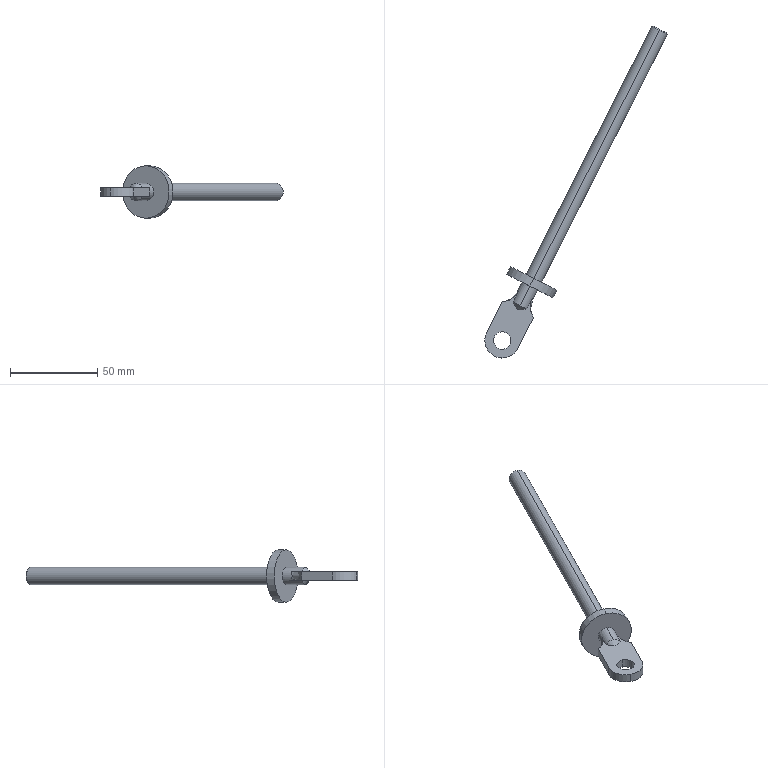Component | SolidWorks | FilmPressingSoilCoveringMechanism2Reverse-2_TieRod2-1 | 1 solid | 24 faces | box 104.65 x 190.43 x 30 mm | volume 19756 mm3 | cylinder 10 | plane 7 | cone 5 | spline 2 | commonest cylinder face diameters 10 x6 30 x2 20 x2
STEP:
#1=COLOUR_RGB('',0.7922,0.8196,0.9333);
#2=FILL_AREA_STYLE_COLOUR('',#1);
#3=FILL_AREA_STYLE('',(#2));
#4=SURFACE_STYLE_FILL_AREA(#3);
#5=SURFACE_SIDE_STYLE('',(#4));
#6=SURFACE_STYLE_USAGE(.BOTH.,#5);
#7=PRESENTATION_STYLE_ASSIGNMENT((#6));
#8=CARTESIAN_POINT('',(-66.242,-3.201,100.924));
#9=VERTEX_POINT('',#8);
#10=CARTESIAN_POINT('',(-66.242,-3.201,101.278));
#11=VERTEX_POINT('',#10);
#12=CARTESIAN_POINT('',(-66.242,-3.201,101.101));
#13=DIRECTION('',(0.4521,0.892,0.));
#14=DIRECTION('',(0.,0.,-1.));
#15=AXIS2_PLACEMENT_3D('',#12,#13,#14);
#16=CIRCLE('',#15,0.1772);
#17=EDGE_CURVE('',#9,#11,#16,.T.);
#18=ORIENTED_EDGE('',*,*,#17,.F.);
#19=CARTESIAN_POINT('',(-66.251,-3.218,100.904));
#20=VERTEX_POINT('',#19);
#21=CARTESIAN_POINT('',(-66.242,-3.201,100.924));
#22=DIRECTION('',(-0.3197,-0.6307,-0.7071));
#23=VECTOR('',#22,39.37);
#24=LINE('',#21,#23);
#25=EDGE_CURVE('',#9,#20,#24,.T.);
#26=ORIENTED_EDGE('',*,*,#25,.T.);
#27=CARTESIAN_POINT('',(-66.251,-3.218,101.298));
#28=VERTEX_POINT('',#27);
#29=CARTESIAN_POINT('',(-66.251,-3.218,101.101));
#30=DIRECTION('',(-0.4521,-0.892,-0.));
#31=DIRECTION('',(0.,0.,-1.));
#32=AXIS2_PLACEMENT_3D('',#29,#30,#31);
#33=CIRCLE('',#32,0.1969);
#34=EDGE_CURVE('',#28,#20,#33,.T.);
#35=ORIENTED_EDGE('',*,*,#34,.F.);
#36=CARTESIAN_POINT('',(-66.242,-3.201,101.278));
#37=DIRECTION('',(-0.3197,-0.6307,0.7071));
#38=VECTOR('',#37,39.37);
#39=LINE('',#36,#38);
#40=EDGE_CURVE('',#11,#28,#39,.T.);
#41=ORIENTED_EDGE('',*,*,#40,.F.);
#42=EDGE_LOOP('',(#18,#26,#35,#41));
#43=FACE_OUTER_BOUND('',#42,.T.);
#44=CARTESIAN_POINT('',(-66.242,-3.201,101.101));
#45=DIRECTION('',(-0.4521,-0.892,-0.));
#46=DIRECTION('',(-0.,-0.,1.));
#47=AXIS2_PLACEMENT_3D('',#44,#45,#46);
#48=CONICAL_SURFACE('',#47,0.1772,0.7854);
#49=ADVANCED_FACE('',(#43),#48,.T.);
#50=CARTESIAN_POINT('',(-69.446,-9.522,101.003));
#51=VERTEX_POINT('',#50);
#52=CARTESIAN_POINT('',(-69.25,-9.511,101.003));
#53=VERTEX_POINT('',#52);
#54=CARTESIAN_POINT('',(-69.446,-9.522,101.003));
#55=CARTESIAN_POINT('',(-69.439,-9.526,101.003));
#56=CARTESIAN_POINT('',(-69.431,-9.528,101.003));
#57=CARTESIAN_POINT('',(-69.415,-9.532,101.003));
#58=CARTESIAN_POINT('',(-69.406,-9.533,101.003));
#59=CARTESIAN_POINT('',(-69.381,-9.534,101.003));
#60=CARTESIAN_POINT('',(-69.364,-9.533,101.003));
#61=CARTESIAN_POINT('',(-69.331,-9.529,101.003));
#62=CARTESIAN_POINT('',(-69.315,-9.526,101.003));
#63=CARTESIAN_POINT('',(-69.282,-9.519,101.003));
#64=CARTESIAN_POINT('',(-69.266,-9.515,101.003));
#65=CARTESIAN_POINT('',(-69.25,-9.511,101.003));
#66=B_SPLINE_CURVE_WITH_KNOTS('',3,(#54,#55,#56,#57,#58,#59,#60,#61,#62,#63,#64,#65),.UNSPECIFIED.,.F.,.F.,(4,2,2,2,2,4),(0.005096,0.005734,0.006372,0.007648,0.008924,0.0102),.UNSPECIFIED.);
#67=EDGE_CURVE('',#51,#53,#66,.T.);
#68=ORIENTED_EDGE('',*,*,#67,.F.);
#69=CARTESIAN_POINT('',(-69.402,-9.434,100.904));
#70=VERTEX_POINT('',#69);
#71=CARTESIAN_POINT('',(-69.402,-9.434,100.904));
#72=DIRECTION('',(0.3197,0.6307,-0.7071));
#73=VECTOR('',#72,39.37);
#74=LINE('',#71,#73);
#75=EDGE_CURVE('',#51,#70,#74,.T.);
#76=ORIENTED_EDGE('',*,*,#75,.T.);
#77=CARTESIAN_POINT('',(-69.402,-9.434,101.101));
#78=DIRECTION('',(0.4521,0.892,0.));
#79=DIRECTION('',(0.,0.,-1.));
#80=AXIS2_PLACEMENT_3D('',#77,#78,#79);
#81=CIRCLE('',#80,0.1969);
#82=EDGE_CURVE('',#53,#70,#81,.T.);
#83=ORIENTED_EDGE('',*,*,#82,.F.);
#84=EDGE_LOOP('',(#68,#76,#83));
#85=FACE_OUTER_BOUND('',#84,.T.);
#86=CARTESIAN_POINT('',(-69.402,-9.434,101.101));
#87=DIRECTION('',(0.4521,0.892,0.));
#88=DIRECTION('',(0.,0.,-1.));
#89=AXIS2_PLACEMENT_3D('',#86,#87,#88);
#90=CONICAL_SURFACE('',#89,0.1969,0.7854);
#91=ADVANCED_FACE('',(#85),#90,.T.);
#92=CARTESIAN_POINT('',(-69.891,-10.4,101.003));
#93=VERTEX_POINT('',#92);
#94=CARTESIAN_POINT('',(-69.713,-10.048,101.003));
#95=VERTEX_POINT('',#94);
#96=CARTESIAN_POINT('',(-69.802,-10.224,101.003));
#97=DIRECTION('',(-0.,-0.,1.));
#98=DIRECTION('',(0.4521,0.892,0.));
#99=AXIS2_PLACEMENT_3D('',#96,#97,#98);
#100=CIRCLE('',#99,0.1969);
#101=EDGE_CURVE('',#93,#95,#100,.T.);
#102=ORIENTED_EDGE('',*,*,#101,.F.);
#103=CARTESIAN_POINT('',(-69.891,-10.4,101.2));
#104=VERTEX_POINT('',#103);
#105=CARTESIAN_POINT('',(-69.891,-10.4,100.019));
#106=DIRECTION('',(-0.,-0.,1.));
#107=VECTOR('',#106,39.37);
#108=LINE('',#105,#107);
#109=EDGE_CURVE('',#93,#104,#108,.T.);
#110=ORIENTED_EDGE('',*,*,#109,.T.);
#111=CARTESIAN_POINT('',(-69.713,-10.048,101.2));
#112=VERTEX_POINT('',#111);
#113=CARTESIAN_POINT('',(-69.802,-10.224,101.2));
#114=DIRECTION('',(-0.,-0.,1.));
#115=DIRECTION('',(0.4521,0.892,0.));
#116=AXIS2_PLACEMENT_3D('',#113,#114,#115);
#117=CIRCLE('',#116,0.1969);
#118=EDGE_CURVE('',#104,#112,#117,.T.);
#119=ORIENTED_EDGE('',*,*,#118,.T.);
#120=CARTESIAN_POINT('',(-69.713,-10.048,100.019));
#121=DIRECTION('',(-0.,-0.,1.));
#122=VECTOR('',#121,39.37);
#123=LINE('',#120,#122);
#124=EDGE_CURVE('',#95,#112,#123,.T.);
#125=ORIENTED_EDGE('',*,*,#124,.F.);
#126=EDGE_LOOP('',(#102,#110,#119,#125));
#127=FACE_OUTER_BOUND('',#126,.T.);
#128=CARTESIAN_POINT('',(-69.802,-10.224,100.019));
#129=DIRECTION('',(-0.,-0.,1.));
#130=DIRECTION('',(0.4521,0.892,0.));
#131=AXIS2_PLACEMENT_3D('',#128,#129,#130);
#132=CYLINDRICAL_SURFACE('',#131,0.1969);
#133=ADVANCED_FACE('',(#127),#132,.F.);
#134=ORIENTED_EDGE('',*,*,#34,.T.);
#135=CARTESIAN_POINT('',(-69.09,-8.819,100.904));
#136=VERTEX_POINT('',#135);
#137=CARTESIAN_POINT('',(-66.242,-3.201,100.904));
#138=DIRECTION('',(-0.4521,-0.892,-0.));
#139=VECTOR('',#138,39.37);
#140=LINE('',#137,#139);
#141=EDGE_CURVE('',#20,#136,#140,.T.);
#142=ORIENTED_EDGE('',*,*,#141,.T.);
#143=CARTESIAN_POINT('',(-69.09,-8.819,101.298));
#144=VERTEX_POINT('',#143);
#145=CARTESIAN_POINT('',(-69.09,-8.819,101.101));
#146=DIRECTION('',(-0.4521,-0.892,-0.));
#147=DIRECTION('',(-0.,-0.,1.));
#148=AXIS2_PLACEMENT_3D('',#145,#146,#147);
#149=CIRCLE('',#148,0.1969);
#150=EDGE_CURVE('',#144,#136,#149,.T.);
#151=ORIENTED_EDGE('',*,*,#150,.F.);
#152=CARTESIAN_POINT('',(-66.242,-3.201,101.298));
#153=DIRECTION('',(-0.4521,-0.892,-0.));
#154=VECTOR('',#153,39.37);
#155=LINE('',#152,#154);
#156=EDGE_CURVE('',#28,#144,#155,.T.);
#157=ORIENTED_EDGE('',*,*,#156,.F.);
#158=EDGE_LOOP('',(#134,#142,#151,#157));
#159=FACE_OUTER_BOUND('',#158,.T.);
#160=CARTESIAN_POINT('',(-66.242,-3.201,101.101));
#161=DIRECTION('',(-0.4521,-0.892,-0.));
#162=DIRECTION('',(-0.,-0.,1.));
#163=AXIS2_PLACEMENT_3D('',#160,#161,#162);
#164=CYLINDRICAL_SURFACE('',#163,0.1969);
#165=ADVANCED_FACE('',(#159),#164,.T.);
#166=CARTESIAN_POINT('',(-69.179,-8.995,101.692));
#167=VERTEX_POINT('',#166);
#168=CARTESIAN_POINT('',(-69.179,-8.995,100.511));
#169=VERTEX_POINT('',#168);
#170=CARTESIAN_POINT('',(-69.179,-8.995,101.101));
#171=DIRECTION('',(-0.4521,-0.892,-0.));
#172=DIRECTION('',(-0.,-0.,1.));
#173=AXIS2_PLACEMENT_3D('',#170,#171,#172);
#174=CIRCLE('',#173,0.5906);
#175=EDGE_CURVE('',#167,#169,#174,.T.);
#176=ORIENTED_EDGE('',*,*,#175,.F.);
#177=CARTESIAN_POINT('',(-69.09,-8.819,101.692));
#178=VERTEX_POINT('',#177);
#179=CARTESIAN_POINT('',(-69.179,-8.995,101.692));
#180=DIRECTION('',(0.4521,0.892,0.));
#181=VECTOR('',#180,39.37);
#182=LINE('',#179,#181);
#183=EDGE_CURVE('',#167,#178,#182,.T.);
#184=ORIENTED_EDGE('',*,*,#183,.T.);
#185=CARTESIAN_POINT('',(-69.09,-8.819,100.511));
#186=VERTEX_POINT('',#185);
#187=CARTESIAN_POINT('',(-69.09,-8.819,101.101));
#188=DIRECTION('',(-0.4521,-0.892,-0.));
#189=DIRECTION('',(-0.,-0.,1.));
#190=AXIS2_PLACEMENT_3D('',#187,#188,#189);
#191=CIRCLE('',#190,0.5906);
#192=EDGE_CURVE('',#178,#186,#191,.T.);
#193=ORIENTED_EDGE('',*,*,#192,.T.);
#194=CARTESIAN_POINT('',(-69.179,-8.995,100.511));
#195=DIRECTION('',(0.4521,0.892,0.));
#196=VECTOR('',#195,39.37);
#197=LINE('',#194,#196);
#198=EDGE_CURVE('',#169,#186,#197,.T.);
#199=ORIENTED_EDGE('',*,*,#198,.F.);
#200=EDGE_LOOP('',(#176,#184,#193,#199));
#201=FACE_OUTER_BOUND('',#200,.T.);
#202=CARTESIAN_POINT('',(-69.179,-8.995,101.101));
#203=DIRECTION('',(0.4521,0.892,0.));
#204=DIRECTION('',(0.,0.,-1.));
#205=AXIS2_PLACEMENT_3D('',#202,#203,#204);
#206=CYLINDRICAL_SURFACE('',#205,0.5906);
#207=ADVANCED_FACE('',(#201),#206,.T.);
#208=CARTESIAN_POINT('',(-69.179,-8.995,101.298));
#209=VERTEX_POINT('',#208);
#210=CARTESIAN_POINT('',(-69.179,-8.995,100.904));
#211=VERTEX_POINT('',#210);
#212=CARTESIAN_POINT('',(-69.179,-8.995,101.101));
#213=DIRECTION('',(-0.4521,-0.892,-0.));
#214=DIRECTION('',(-0.,-0.,1.));
#215=AXIS2_PLACEMENT_3D('',#212,#213,#214);
#216=CIRCLE('',#215,0.1969);
#217=EDGE_CURVE('',#209,#211,#216,.T.);
#218=ORIENTED_EDGE('',*,*,#217,.T.);
#219=CARTESIAN_POINT('',(-66.242,-3.201,100.904));
#220=DIRECTION('',(-0.4521,-0.892,-0.));
#221=VECTOR('',#220,39.37);
#222=LINE('',#219,#221);
#223=EDGE_CURVE('',#211,#70,#222,.T.);
#224=ORIENTED_EDGE('',*,*,#223,.T.);
#225=CARTESIAN_POINT('',(-69.554,-9.357,101.003));
#226=VERTEX_POINT('',#225);
#227=CARTESIAN_POINT('',(-69.402,-9.434,101.101));
#228=DIRECTION('',(0.4521,0.892,0.));
#229=DIRECTION('',(0.,0.,-1.));
#230=AXIS2_PLACEMENT_3D('',#227,#228,#229);
#231=CIRCLE('',#230,0.1969);
#232=EDGE_CURVE('',#70,#226,#231,.T.);
#233=ORIENTED_EDGE('',*,*,#232,.T.);
#234=CARTESIAN_POINT('',(-69.429,-9.11,101.003));
#235=VERTEX_POINT('',#234);
#236=CARTESIAN_POINT('',(-69.598,-9.445,101.003));
#237=DIRECTION('',(0.4521,0.892,0.));
#238=VECTOR('',#237,39.37);
#239=LINE('',#236,#238);
#240=EDGE_CURVE('',#226,#235,#239,.T.);
#241=ORIENTED_EDGE('',*,*,#240,.T.);
#242=CARTESIAN_POINT('',(-69.429,-9.11,101.2));
#243=VERTEX_POINT('',#242);
#244=CARTESIAN_POINT('',(-69.429,-9.11,101.003));
#245=CARTESIAN_POINT('',(-69.434,-9.111,101.01));
#246=CARTESIAN_POINT('',(-69.439,-9.113,101.017));
#247=CARTESIAN_POINT('',(-69.448,-9.117,101.033));
#248=CARTESIAN_POINT('',(-69.453,-9.12,101.04));
#249=CARTESIAN_POINT('',(-69.46,-9.124,101.057));
#250=CARTESIAN_POINT('',(-69.463,-9.125,101.065));
#251=CARTESIAN_POINT('',(-69.467,-9.128,101.083));
#252=CARTESIAN_POINT('',(-69.468,-9.129,101.092));
#253=CARTESIAN_POINT('',(-69.468,-9.129,101.106));
#254=CARTESIAN_POINT('',(-69.467,-9.128,101.11));
#255=CARTESIAN_POINT('',(-69.466,-9.128,101.12));
#256=CARTESIAN_POINT('',(-69.466,-9.127,101.124));
#257=CARTESIAN_POINT('',(-69.463,-9.125,101.137));
#258=CARTESIAN_POINT('',(-69.46,-9.124,101.146));
#259=CARTESIAN_POINT('',(-69.449,-9.118,101.17));
#260=CARTESIAN_POINT('',(-69.439,-9.113,101.185));
#261=CARTESIAN_POINT('',(-69.429,-9.11,101.2));
#262=B_SPLINE_CURVE_WITH_KNOTS('',3,(#244,#245,#246,#247,#248,#249,#250,#251,#252,#253,#254,#255,#256,#257,#258,#259,#260,#261),.UNSPECIFIED.,.F.,.F.,(4,2,2,2,2,2,2,2,4),(0.,0.0006968,0.001394,0.00209,0.002787,0.003135,0.003484,0.004181,0.005574),.UNSPECIFIED.);
#263=EDGE_CURVE('',#235,#243,#262,.T.);
#264=ORIENTED_EDGE('',*,*,#263,.T.);
#265=CARTESIAN_POINT('',(-69.554,-9.357,101.2));
#266=VERTEX_POINT('',#265);
#267=CARTESIAN_POINT('',(-69.429,-9.11,101.2));
#268=DIRECTION('',(-0.4521,-0.892,-0.));
#269=VECTOR('',#268,39.37);
#270=LINE('',#267,#269);
#271=EDGE_CURVE('',#243,#266,#270,.T.);
#272=ORIENTED_EDGE('',*,*,#271,.T.);
#273=CARTESIAN_POINT('',(-69.402,-9.434,101.298));
#274=VERTEX_POINT('',#273);
#275=CARTESIAN_POINT('',(-69.402,-9.434,101.101));
#276=DIRECTION('',(0.4521,0.892,0.));
#277=DIRECTION('',(0.,0.,-1.));
#278=AXIS2_PLACEMENT_3D('',#275,#276,#277);
#279=CIRCLE('',#278,0.1969);
#280=EDGE_CURVE('',#266,#274,#279,.T.);
#281=ORIENTED_EDGE('',*,*,#280,.T.);
#282=CARTESIAN_POINT('',(-66.242,-3.201,101.298));
#283=DIRECTION('',(-0.4521,-0.892,-0.));
#284=VECTOR('',#283,39.37);
#285=LINE('',#282,#284);
#286=EDGE_CURVE('',#209,#274,#285,.T.);
#287=ORIENTED_EDGE('',*,*,#286,.F.);
#288=EDGE_LOOP('',(#218,#224,#233,#241,#264,#272,#281,#287));
#289=FACE_OUTER_BOUND('',#288,.T.);
#290=CARTESIAN_POINT('',(-66.242,-3.201,101.101));
#291=DIRECTION('',(-0.4521,-0.892,-0.));
#292=DIRECTION('',(-0.,-0.,1.));
#293=AXIS2_PLACEMENT_3D('',#290,#291,#292);
#294=CYLINDRICAL_SURFACE('',#293,0.1969);
#295=ADVANCED_FACE('',(#289),#294,.T.);
#296=ORIENTED_EDGE('',*,*,#223,.F.);
#297=CARTESIAN_POINT('',(-69.179,-8.995,101.101));
#298=DIRECTION('',(-0.4521,-0.892,-0.));
#299=DIRECTION('',(-0.,-0.,1.));
#300=AXIS2_PLACEMENT_3D('',#297,#298,#299);
#301=CIRCLE('',#300,0.1969);
#302=EDGE_CURVE('',#211,#209,#301,.T.);
#303=ORIENTED_EDGE('',*,*,#302,.T.);
#304=ORIENTED_EDGE('',*,*,#286,.T.);
#305=CARTESIAN_POINT('',(-69.25,-9.511,101.2));
#306=VERTEX_POINT('',#305);
#307=CARTESIAN_POINT('',(-69.402,-9.434,101.101));
#308=DIRECTION('',(0.4521,0.892,0.));
#309=DIRECTION('',(0.,0.,-1.));
#310=AXIS2_PLACEMENT_3D('',#307,#308,#309);
#311=CIRCLE('',#310,0.1969);
#312=EDGE_CURVE('',#274,#306,#311,.T.);
#313=ORIENTED_EDGE('',*,*,#312,.T.);
#314=CARTESIAN_POINT('',(-69.124,-9.264,101.2));
#315=VERTEX_POINT('',#314);
#316=CARTESIAN_POINT('',(-69.294,-9.599,101.2));
#317=DIRECTION('',(0.4521,0.892,0.));
#318=VECTOR('',#317,39.37);
#319=LINE('',#316,#318);
#320=EDGE_CURVE('',#306,#315,#319,.T.);
#321=ORIENTED_EDGE('',*,*,#320,.T.);
#322=CARTESIAN_POINT('',(-69.124,-9.264,101.003));
#323=VERTEX_POINT('',#322);
#324=CARTESIAN_POINT('',(-69.124,-9.264,101.2));
#325=CARTESIAN_POINT('',(-69.122,-9.269,101.192));
#326=CARTESIAN_POINT('',(-69.121,-9.274,101.185));
#327=CARTESIAN_POINT('',(-69.119,-9.284,101.17));
#328=CARTESIAN_POINT('',(-69.118,-9.289,101.162));
#329=CARTESIAN_POINT('',(-69.117,-9.297,101.146));
#330=CARTESIAN_POINT('',(-69.117,-9.301,101.137));
#331=CARTESIAN_POINT('',(-69.117,-9.305,101.12));
#332=CARTESIAN_POINT('',(-69.117,-9.307,101.11));
#333=CARTESIAN_POINT('',(-69.117,-9.307,101.097));
#334=CARTESIAN_POINT('',(-69.117,-9.306,101.092));
#335=CARTESIAN_POINT('',(-69.117,-9.305,101.083));
#336=CARTESIAN_POINT('',(-69.117,-9.304,101.078));
#337=CARTESIAN_POINT('',(-69.117,-9.301,101.065));
#338=CARTESIAN_POINT('',(-69.117,-9.297,101.057));
#339=CARTESIAN_POINT('',(-69.119,-9.285,101.032));
#340=CARTESIAN_POINT('',(-69.121,-9.274,101.017));
#341=CARTESIAN_POINT('',(-69.124,-9.264,101.003));
#342=B_SPLINE_CURVE_WITH_KNOTS('',3,(#324,#325,#326,#327,#328,#329,#330,#331,#332,#333,#334,#335,#336,#337,#338,#339,#340,#341),.UNSPECIFIED.,.F.,.F.,(4,2,2,2,2,2,2,2,4),(0.,0.0006968,0.001394,0.00209,0.002787,0.003135,0.003484,0.004181,0.005574),.UNSPECIFIED.);
#343=EDGE_CURVE('',#315,#323,#342,.T.);
#344=ORIENTED_EDGE('',*,*,#343,.T.);
#345=CARTESIAN_POINT('',(-69.124,-9.264,101.003));
#346=DIRECTION('',(-0.4521,-0.892,-0.));
#347=VECTOR('',#346,39.37);
#348=LINE('',#345,#347);
#349=EDGE_CURVE('',#323,#53,#348,.T.);
#350=ORIENTED_EDGE('',*,*,#349,.T.);
#351=ORIENTED_EDGE('',*,*,#82,.T.);
#352=EDGE_LOOP('',(#296,#303,#304,#313,#321,#344,#350,#351));
#353=FACE_OUTER_BOUND('',#352,.T.);
#354=CARTESIAN_POINT('',(-66.242,-3.201,101.101));
#355=DIRECTION('',(-0.4521,-0.892,-0.));
#356=DIRECTION('',(-0.,-0.,1.));
#357=AXIS2_PLACEMENT_3D('',#354,#355,#356);
#358=CYLINDRICAL_SURFACE('',#357,0.1969);
#359=ADVANCED_FACE('',(#353),#358,.T.);
#360=CARTESIAN_POINT('',(-69.179,-8.995,101.101));
#361=DIRECTION('',(-0.4521,-0.892,-0.));
#362=DIRECTION('',(-0.,-0.,1.));
#363=AXIS2_PLACEMENT_3D('',#360,#361,#362);
#364=CIRCLE('',#363,0.5906);
#365=EDGE_CURVE('',#169,#167,#364,.T.);
#366=ORIENTED_EDGE('',*,*,#365,.T.);
#367=ORIENTED_EDGE('',*,*,#175,.T.);
#368=EDGE_LOOP('',(#366,#367));
#369=FACE_OUTER_BOUND('',#368,.T.);
#370=ORIENTED_EDGE('',*,*,#217,.F.);
#371=ORIENTED_EDGE('',*,*,#302,.F.);
#372=EDGE_LOOP('',(#370,#371));
#373=FACE_BOUND('',#372,.T.);
#374=CARTESIAN_POINT('',(-69.179,-8.995,101.101));
#375=DIRECTION('',(-0.4521,-0.892,-0.));
#376=DIRECTION('',(-0.,-0.,1.));
#377=AXIS2_PLACEMENT_3D('',#374,#375,#376);
#378=PLANE('',#377);
#379=ADVANCED_FACE('',(#369,#373),#378,.T.);
#380=CARTESIAN_POINT('',(-69.09,-8.819,101.101));
#381=DIRECTION('',(-0.4521,-0.892,-0.));
#382=DIRECTION('',(-0.,-0.,1.));
#383=AXIS2_PLACEMENT_3D('',#380,#381,#382);
#384=CIRCLE('',#383,0.5906);
#385=EDGE_CURVE('',#186,#178,#384,.T.);
#386=ORIENTED_EDGE('',*,*,#385,.F.);
#387=ORIENTED_EDGE('',*,*,#192,.F.);
#388=EDGE_LOOP('',(#386,#387));
#389=FACE_OUTER_BOUND('',#388,.T.);
#390=ORIENTED_EDGE('',*,*,#150,.T.);
#391=CARTESIAN_POINT('',(-69.09,-8.819,101.101));
#392=DIRECTION('',(-0.4521,-0.892,-0.));
#393=DIRECTION('',(-0.,-0.,1.));
#394=AXIS2_PLACEMENT_3D('',#391,#392,#393);
#395=CIRCLE('',#394,0.1969);
#396=EDGE_CURVE('',#136,#144,#395,.T.);
#397=ORIENTED_EDGE('',*,*,#396,.T.);
#398=EDGE_LOOP('',(#390,#397));
#399=FACE_BOUND('',#398,.T.);
#400=CARTESIAN_POINT('',(-69.09,-8.819,101.101));
#401=DIRECTION('',(-0.4521,-0.892,-0.));
#402=DIRECTION('',(-0.,-0.,1.));
#403=AXIS2_PLACEMENT_3D('',#400,#401,#402);
#404=PLANE('',#403);
#405=ADVANCED_FACE('',(#389,#399),#404,.F.);
#406=ORIENTED_EDGE('',*,*,#183,.F.);
#407=ORIENTED_EDGE('',*,*,#365,.F.);
#408=ORIENTED_EDGE('',*,*,#198,.T.);
#409=ORIENTED_EDGE('',*,*,#385,.T.);
#410=EDGE_LOOP('',(#406,#407,#408,#409));
#411=FACE_OUTER_BOUND('',#410,.T.);
#412=CARTESIAN_POINT('',(-69.179,-8.995,101.101));
#413=DIRECTION('',(0.4521,0.892,0.));
#414=DIRECTION('',(0.,0.,-1.));
#415=AXIS2_PLACEMENT_3D('',#412,#413,#414);
#416=CYLINDRICAL_SURFACE('',#415,0.5906);
#417=ADVANCED_FACE('',(#411),#416,.T.);
#418=CARTESIAN_POINT('',(-66.242,-3.201,101.101));
#419=DIRECTION('',(0.4521,0.892,0.));
#420=DIRECTION('',(0.,0.,-1.));
#421=AXIS2_PLACEMENT_3D('',#418,#419,#420);
#422=CIRCLE('',#421,0.1772);
#423=EDGE_CURVE('',#11,#9,#422,.T.);
#424=ORIENTED_EDGE('',*,*,#423,.T.);
#425=ORIENTED_EDGE('',*,*,#17,.T.);
#426=EDGE_LOOP('',(#424,#425));
#427=FACE_OUTER_BOUND('',#426,.T.);
#428=CARTESIAN_POINT('',(-66.242,-3.201,101.101));
#429=DIRECTION('',(0.4521,0.892,0.));
#430=DIRECTION('',(0.,0.,-1.));
#431=AXIS2_PLACEMENT_3D('',#428,#429,#430);
#432=PLANE('',#431);
#433=ADVANCED_FACE('',(#427),#432,.T.);
#434=ORIENTED_EDGE('',*,*,#141,.F.);
#435=CARTESIAN_POINT('',(-66.251,-3.218,101.101));
#436=DIRECTION('',(-0.4521,-0.892,-0.));
#437=DIRECTION('',(0.,0.,-1.));
#438=AXIS2_PLACEMENT_3D('',#435,#436,#437);
#439=CIRCLE('',#438,0.1969);
#440=EDGE_CURVE('',#20,#28,#439,.T.);
#441=ORIENTED_EDGE('',*,*,#440,.T.);
#442=ORIENTED_EDGE('',*,*,#156,.T.);
#443=ORIENTED_EDGE('',*,*,#396,.F.);
#444=EDGE_LOOP('',(#434,#441,#442,#443));
#445=FACE_OUTER_BOUND('',#444,.T.);
#446=CARTESIAN_POINT('',(-66.242,-3.201,101.101));
#447=DIRECTION('',(-0.4521,-0.892,-0.));
#448=DIRECTION('',(-0.,-0.,1.));
#449=AXIS2_PLACEMENT_3D('',#446,#447,#448);
#450=CYLINDRICAL_SURFACE('',#449,0.1969);
#451=ADVANCED_FACE('',(#445),#450,.T.);
#452=CARTESIAN_POINT('',(-69.802,-10.224,101.2));
#453=DIRECTION('',(-0.,-0.,1.));
#454=DIRECTION('',(0.4521,0.892,0.));
#455=AXIS2_PLACEMENT_3D('',#452,#453,#454);
#456=CIRCLE('',#455,0.1969);
#457=EDGE_CURVE('',#112,#104,#456,.T.);
#458=ORIENTED_EDGE('',*,*,#457,.F.);
#459=ORIENTED_EDGE('',*,*,#118,.F.);
#460=EDGE_LOOP('',(#458,#459));
#461=FACE_BOUND('',#460,.T.);
#462=CARTESIAN_POINT('',(-70.153,-10.046,101.2));
#463=VERTEX_POINT('',#462);
#464=CARTESIAN_POINT('',(-69.797,-9.344,101.2));
#465=VERTEX_POINT('',#464);
#466=CARTESIAN_POINT('',(-70.331,-10.397,101.2));
#467=DIRECTION('',(0.4521,0.892,0.));
#468=VECTOR('',#467,39.37);
#469=LINE('',#466,#468);
#470=EDGE_CURVE('',#463,#465,#469,.T.);
#471=ORIENTED_EDGE('',*,*,#470,.F.);
#472=CARTESIAN_POINT('',(-69.98,-10.575,101.2));
#473=VERTEX_POINT('',#472);
#474=CARTESIAN_POINT('',(-69.802,-10.224,101.2));
#475=DIRECTION('',(-0.,-0.,1.));
#476=DIRECTION('',(-0.4521,-0.892,-0.));
#477=AXIS2_PLACEMENT_3D('',#474,#475,#476);
#478=CIRCLE('',#477,0.3937);
#479=EDGE_CURVE('',#463,#473,#478,.T.);
#480=ORIENTED_EDGE('',*,*,#479,.T.);
#481=CARTESIAN_POINT('',(-69.451,-10.402,101.2));
#482=VERTEX_POINT('',#481);
#483=CARTESIAN_POINT('',(-69.802,-10.224,101.2));
#484=DIRECTION('',(-0.,-0.,1.));
#485=DIRECTION('',(-0.4521,-0.892,-0.));
#486=AXIS2_PLACEMENT_3D('',#483,#484,#485);
#487=CIRCLE('',#486,0.3937);
#488=EDGE_CURVE('',#473,#482,#487,.T.);
#489=ORIENTED_EDGE('',*,*,#488,.T.);
#490=CARTESIAN_POINT('',(-69.095,-9.7,101.2));
#491=VERTEX_POINT('',#490);
#492=CARTESIAN_POINT('',(-69.629,-10.753,101.2));
#493=DIRECTION('',(0.4521,0.892,0.));
#494=VECTOR('',#493,39.37);
#495=LINE('',#492,#494);
#496=EDGE_CURVE('',#482,#491,#495,.T.);
#497=ORIENTED_EDGE('',*,*,#496,.T.);
#498=CARTESIAN_POINT('',(-69.095,-9.7,101.2));
#499=CARTESIAN_POINT('',(-69.117,-9.668,101.2));
#500=CARTESIAN_POINT('',(-69.134,-9.634,101.2));
#501=CARTESIAN_POINT('',(-69.152,-9.58,101.2));
#502=CARTESIAN_POINT('',(-69.157,-9.561,101.2));
#503=CARTESIAN_POINT('',(-69.164,-9.524,101.2));
#504=CARTESIAN_POINT('',(-69.167,-9.505,101.2));
#505=CARTESIAN_POINT('',(-69.169,-9.467,101.2));
#506=CARTESIAN_POINT('',(-69.169,-9.448,101.2));
#507=CARTESIAN_POINT('',(-69.167,-9.409,101.2));
#508=CARTESIAN_POINT('',(-69.164,-9.391,101.2));
#509=CARTESIAN_POINT('',(-69.157,-9.353,101.2));
#510=CARTESIAN_POINT('',(-69.152,-9.335,101.2));
#511=CARTESIAN_POINT('',(-69.14,-9.299,101.2));
#512=CARTESIAN_POINT('',(-69.133,-9.281,101.2));
#513=CARTESIAN_POINT('',(-69.124,-9.264,101.2));
#514=B_SPLINE_CURVE_WITH_KNOTS('',3,(#498,#499,#500,#501,#502,#503,#504,#505,#506,#507,#508,#509,#510,#511,#512,#513),.UNSPECIFIED.,.F.,.F.,(4,2,2,2,2,2,2,4),(0.,0.002891,0.004336,0.005781,0.007227,0.008672,0.01012,0.01156),.UNSPECIFIED.);
#515=EDGE_CURVE('',#491,#315,#514,.T.);
#516=ORIENTED_EDGE('',*,*,#515,.T.);
#517=ORIENTED_EDGE('',*,*,#320,.F.);
#518=CARTESIAN_POINT('',(-69.25,-9.511,101.2));
#519=CARTESIAN_POINT('',(-69.266,-9.515,101.2));
#520=CARTESIAN_POINT('',(-69.282,-9.519,101.2));
#521=CARTESIAN_POINT('',(-69.315,-9.526,101.2));
#522=CARTESIAN_POINT('',(-69.332,-9.529,101.2));
#523=CARTESIAN_POINT('',(-69.365,-9.533,101.2));
#524=CARTESIAN_POINT('',(-69.381,-9.534,101.2));
#525=CARTESIAN_POINT('',(-69.407,-9.533,101.2));
#526=CARTESIAN_POINT('',(-69.415,-9.532,101.2));
#527=CARTESIAN_POINT('',(-69.431,-9.528,101.2));
#528=CARTESIAN_POINT('',(-69.439,-9.525,101.2));
#529=CARTESIAN_POINT('',(-69.454,-9.518,101.2));
#530=CARTESIAN_POINT('',(-69.461,-9.513,101.2));
#531=CARTESIAN_POINT('',(-69.474,-9.502,101.2));
#532=CARTESIAN_POINT('',(-69.479,-9.496,101.2));
#533=CARTESIAN_POINT('',(-69.495,-9.477,101.2));
#534=CARTESIAN_POINT('',(-69.504,-9.462,101.2));
#535=CARTESIAN_POINT('',(-69.52,-9.433,101.2));
#536=CARTESIAN_POINT('',(-69.527,-9.418,101.2));
#537=CARTESIAN_POINT('',(-69.541,-9.388,101.2));
#538=CARTESIAN_POINT('',(-69.548,-9.372,101.2));
#539=CARTESIAN_POINT('',(-69.554,-9.357,101.2));
#540=B_SPLINE_CURVE_WITH_KNOTS('',3,(#518,#519,#520,#521,#522,#523,#524,#525,#526,#527,#528,#529,#530,#531,#532,#533,#534,#535,#536,#537,#538,#539),.UNSPECIFIED.,.F.,.F.,(4,2,2,2,2,2,2,2,2,2,4),(0.,0.001275,0.00255,0.003825,0.004463,0.0051,0.005738,0.006375,0.00765,0.008925,0.0102),.UNSPECIFIED.);
#541=EDGE_CURVE('',#306,#266,#540,.T.);
#542=ORIENTED_EDGE('',*,*,#541,.T.);
#543=ORIENTED_EDGE('',*,*,#271,.F.);
#544=CARTESIAN_POINT('',(-69.429,-9.11,101.2));
#545=CARTESIAN_POINT('',(-69.437,-9.127,101.2));
#546=CARTESIAN_POINT('',(-69.447,-9.143,101.2));
#547=CARTESIAN_POINT('',(-69.469,-9.174,101.2));
#548=CARTESIAN_POINT('',(-69.481,-9.189,101.2));
#549=CARTESIAN_POINT('',(-69.507,-9.217,101.2));
#550=CARTESIAN_POINT('',(-69.521,-9.23,101.2));
#551=CARTESIAN_POINT('',(-69.55,-9.255,101.2));
#552=CARTESIAN_POINT('',(-69.566,-9.266,101.2));
#553=CARTESIAN_POINT('',(-69.598,-9.286,101.2));
#554=CARTESIAN_POINT('',(-69.614,-9.296,101.2));
#555=CARTESIAN_POINT('',(-69.649,-9.312,101.2));
#556=CARTESIAN_POINT('',(-69.667,-9.319,101.2));
#557=CARTESIAN_POINT('',(-69.703,-9.33,101.2));
#558=CARTESIAN_POINT('',(-69.722,-9.335,101.2));
#559=CARTESIAN_POINT('',(-69.759,-9.341,101.2));
#560=CARTESIAN_POINT('',(-69.778,-9.343,101.2));
#561=CARTESIAN_POINT('',(-69.797,-9.344,101.2));
#562=B_SPLINE_CURVE_WITH_KNOTS('',3,(#544,#545,#546,#547,#548,#549,#550,#551,#552,#553,#554,#555,#556,#557,#558,#559,#560,#561),.UNSPECIFIED.,.F.,.F.,(4,2,2,2,2,2,2,2,4),(0.,0.001446,0.002892,0.004338,0.005784,0.00723,0.008676,0.01012,0.01157),.UNSPECIFIED.);
#563=EDGE_CURVE('',#243,#465,#562,.T.);
#564=ORIENTED_EDGE('',*,*,#563,.T.);
#565=EDGE_LOOP('',(#471,#480,#489,#497,#516,#517,#542,#543,#564));
#566=FACE_OUTER_BOUND('',#565,.T.);
#567=CARTESIAN_POINT('',(-69.629,-10.753,101.2));
#568=DIRECTION('',(0.,0.,-1.));
#569=DIRECTION('',(-0.4521,-0.892,-0.));
#570=AXIS2_PLACEMENT_3D('',#567,#568,#569);
#571=PLANE('',#570);
#572=ADVANCED_FACE('',(#461,#566),#571,.F.);
#573=CARTESIAN_POINT('',(-70.153,-10.046,101.003));
#574=VERTEX_POINT('',#573);
#575=CARTESIAN_POINT('',(-69.797,-9.344,101.003));
#576=VERTEX_POINT('',#575);
#577=CARTESIAN_POINT('',(-70.331,-10.397,101.003));
#578=DIRECTION('',(0.4521,0.892,0.));
#579=VECTOR('',#578,39.37);
#580=LINE('',#577,#579);
#581=EDGE_CURVE('',#574,#576,#580,.T.);
#582=ORIENTED_EDGE('',*,*,#581,.F.);
#583=CARTESIAN_POINT('',(-70.153,-10.046,101.003));
#584=DIRECTION('',(-0.,-0.,1.));
#585=VECTOR('',#584,39.37);
#586=LINE('',#583,#585);
#587=EDGE_CURVE('',#574,#463,#586,.T.);
#588=ORIENTED_EDGE('',*,*,#587,.T.);
#589=ORIENTED_EDGE('',*,*,#470,.T.);
#590=CARTESIAN_POINT('',(-69.797,-9.344,101.003));
#591=DIRECTION('',(0.,0.,-1.));
#592=VECTOR('',#591,39.37);
#593=LINE('',#590,#592);
#594=EDGE_CURVE('',#465,#576,#593,.T.);
#595=ORIENTED_EDGE('',*,*,#594,.T.);
#596=EDGE_LOOP('',(#582,#588,#589,#595));
#597=FACE_OUTER_BOUND('',#596,.T.);
#598=CARTESIAN_POINT('',(-70.331,-10.397,101.003));
#599=DIRECTION('',(0.892,-0.4521,-0.));
#600=DIRECTION('',(-0.4521,-0.892,-0.));
#601=AXIS2_PLACEMENT_3D('',#598,#599,#600);
#602=PLANE('',#601);
#603=ADVANCED_FACE('',(#597),#602,.F.);
#604=CARTESIAN_POINT('',(-69.802,-10.224,101.003));
#605=DIRECTION('',(-0.,-0.,1.));
#606=DIRECTION('',(0.4521,0.892,0.));
#607=AXIS2_PLACEMENT_3D('',#604,#605,#606);
#608=CIRCLE('',#607,0.1969);
#609=EDGE_CURVE('',#95,#93,#608,.T.);
#610=ORIENTED_EDGE('',*,*,#609,.T.);
#611=ORIENTED_EDGE('',*,*,#101,.T.);
#612=EDGE_LOOP('',(#610,#611));
#613=FACE_BOUND('',#612,.T.);
#614=CARTESIAN_POINT('',(-69.451,-10.402,101.003));
#615=VERTEX_POINT('',#614);
#616=CARTESIAN_POINT('',(-69.98,-10.575,101.003));
#617=VERTEX_POINT('',#616);
#618=CARTESIAN_POINT('',(-69.802,-10.224,101.003));
#619=DIRECTION('',(0.,0.,-1.));
#620=DIRECTION('',(0.4521,0.892,0.));
#621=AXIS2_PLACEMENT_3D('',#618,#619,#620);
#622=CIRCLE('',#621,0.3937);
#623=EDGE_CURVE('',#615,#617,#622,.T.);
#624=ORIENTED_EDGE('',*,*,#623,.T.);
#625=CARTESIAN_POINT('',(-69.802,-10.224,101.003));
#626=DIRECTION('',(0.,0.,-1.));
#627=DIRECTION('',(0.4521,0.892,0.));
#628=AXIS2_PLACEMENT_3D('',#625,#626,#627);
#629=CIRCLE('',#628,0.3937);
#630=EDGE_CURVE('',#617,#574,#629,.T.);
#631=ORIENTED_EDGE('',*,*,#630,.T.);
#632=ORIENTED_EDGE('',*,*,#581,.T.);
#633=CARTESIAN_POINT('',(-69.797,-9.344,101.003));
#634=CARTESIAN_POINT('',(-69.759,-9.343,101.003));
#635=CARTESIAN_POINT('',(-69.722,-9.336,101.003));
#636=CARTESIAN_POINT('',(-69.667,-9.319,101.003));
#637=CARTESIAN_POINT('',(-69.649,-9.312,101.003));
#638=CARTESIAN_POINT('',(-69.614,-9.296,101.003));
#639=CARTESIAN_POINT('',(-69.598,-9.286,101.003));
#640=CARTESIAN_POINT('',(-69.566,-9.266,101.003));
#641=CARTESIAN_POINT('',(-69.55,-9.255,101.003));
#642=CARTESIAN_POINT('',(-69.521,-9.23,101.003));
#643=CARTESIAN_POINT('',(-69.507,-9.217,101.003));
#644=CARTESIAN_POINT('',(-69.481,-9.189,101.003));
#645=CARTESIAN_POINT('',(-69.469,-9.174,101.003));
#646=CARTESIAN_POINT('',(-69.447,-9.143,101.003));
#647=CARTESIAN_POINT('',(-69.437,-9.127,101.003));
#648=CARTESIAN_POINT('',(-69.429,-9.11,101.003));
#649=B_SPLINE_CURVE_WITH_KNOTS('',3,(#633,#634,#635,#636,#637,#638,#639,#640,#641,#642,#643,#644,#645,#646,#647,#648),.UNSPECIFIED.,.F.,.F.,(4,2,2,2,2,2,2,4),(0.,0.002891,0.004336,0.005781,0.007227,0.008672,0.01012,0.01156),.UNSPECIFIED.);
#650=EDGE_CURVE('',#576,#235,#649,.T.);
#651=ORIENTED_EDGE('',*,*,#650,.T.);
#652=ORIENTED_EDGE('',*,*,#240,.F.);
#653=CARTESIAN_POINT('',(-69.554,-9.357,101.003));
#654=CARTESIAN_POINT('',(-69.548,-9.372,101.003));
#655=CARTESIAN_POINT('',(-69.541,-9.388,101.003));
#656=CARTESIAN_POINT('',(-69.527,-9.418,101.003));
#657=CARTESIAN_POINT('',(-69.52,-9.433,101.003));
#658=CARTESIAN_POINT('',(-69.504,-9.463,101.003));
#659=CARTESIAN_POINT('',(-69.495,-9.477,101.003));
#660=CARTESIAN_POINT('',(-69.479,-9.496,101.003));
#661=CARTESIAN_POINT('',(-69.473,-9.502,101.003));
#662=CARTESIAN_POINT('',(-69.461,-9.513,101.003));
#663=CARTESIAN_POINT('',(-69.454,-9.518,101.003));
#664=CARTESIAN_POINT('',(-69.446,-9.522,101.003));
#665=B_SPLINE_CURVE_WITH_KNOTS('',3,(#653,#654,#655,#656,#657,#658,#659,#660,#661,#662,#663,#664),.UNSPECIFIED.,.F.,.F.,(4,2,2,2,2,4),(0.,0.001274,0.002548,0.003822,0.004459,0.005096),.UNSPECIFIED.);
#666=EDGE_CURVE('',#226,#51,#665,.T.);
#667=ORIENTED_EDGE('',*,*,#666,.T.);
#668=ORIENTED_EDGE('',*,*,#67,.T.);
#669=ORIENTED_EDGE('',*,*,#349,.F.);
#670=CARTESIAN_POINT('',(-69.095,-9.7,101.003));
#671=VERTEX_POINT('',#670);
#672=CARTESIAN_POINT('',(-69.124,-9.264,101.003));
#673=CARTESIAN_POINT('',(-69.133,-9.281,101.003));
#674=CARTESIAN_POINT('',(-69.14,-9.299,101.003));
#675=CARTESIAN_POINT('',(-69.152,-9.335,101.003));
#676=CARTESIAN_POINT('',(-69.157,-9.353,101.003));
#677=CARTESIAN_POINT('',(-69.164,-9.39,101.003));
#678=CARTESIAN_POINT('',(-69.167,-9.41,101.003));
#679=CARTESIAN_POINT('',(-69.169,-9.448,101.003));
#680=CARTESIAN_POINT('',(-69.169,-9.467,101.003));
#681=CARTESIAN_POINT('',(-69.167,-9.505,101.003));
#682=CARTESIAN_POINT('',(-69.165,-9.524,101.003));
#683=CARTESIAN_POINT('',(-69.157,-9.561,101.003));
#684=CARTESIAN_POINT('',(-69.152,-9.58,101.003));
#685=CARTESIAN_POINT('',(-69.14,-9.616,101.003));
#686=CARTESIAN_POINT('',(-69.133,-9.633,101.003));
#687=CARTESIAN_POINT('',(-69.116,-9.667,101.003));
#688=CARTESIAN_POINT('',(-69.106,-9.684,101.003));
#689=CARTESIAN_POINT('',(-69.095,-9.7,101.003));
#690=B_SPLINE_CURVE_WITH_KNOTS('',3,(#672,#673,#674,#675,#676,#677,#678,#679,#680,#681,#682,#683,#684,#685,#686,#687,#688,#689),.UNSPECIFIED.,.F.,.F.,(4,2,2,2,2,2,2,2,4),(0.,0.001446,0.002892,0.004338,0.005784,0.00723,0.008676,0.01012,0.01157),.UNSPECIFIED.);
#691=EDGE_CURVE('',#323,#671,#690,.T.);
#692=ORIENTED_EDGE('',*,*,#691,.T.);
#693=CARTESIAN_POINT('',(-69.629,-10.753,101.003));
#694=DIRECTION('',(0.4521,0.892,0.));
#695=VECTOR('',#694,39.37);
#696=LINE('',#693,#695);
#697=EDGE_CURVE('',#615,#671,#696,.T.);
#698=ORIENTED_EDGE('',*,*,#697,.F.);
#699=EDGE_LOOP('',(#624,#631,#632,#651,#652,#667,#668,#669,#692,#698));
#700=FACE_OUTER_BOUND('',#699,.T.);
#701=CARTESIAN_POINT('',(-69.629,-10.753,101.003));
#702=DIRECTION('',(-0.,-0.,1.));
#703=DIRECTION('',(0.4521,0.892,0.));
#704=AXIS2_PLACEMENT_3D('',#701,#702,#703);
#705=PLANE('',#704);
#706=ADVANCED_FACE('',(#613,#700),#705,.F.);
#707=ORIENTED_EDGE('',*,*,#496,.F.);
#708=CARTESIAN_POINT('',(-69.451,-10.402,101.003));
#709=DIRECTION('',(0.,0.,-1.));
#710=VECTOR('',#709,39.37);
#711=LINE('',#708,#710);
#712=EDGE_CURVE('',#482,#615,#711,.T.);
#713=ORIENTED_EDGE('',*,*,#712,.T.);
#714=ORIENTED_EDGE('',*,*,#697,.T.);
#715=CARTESIAN_POINT('',(-69.095,-9.7,101.003));
#716=DIRECTION('',(-0.,-0.,1.));
#717=VECTOR('',#716,39.37);
#718=LINE('',#715,#717);
#719=EDGE_CURVE('',#671,#491,#718,.T.);
#720=ORIENTED_EDGE('',*,*,#719,.T.);
#721=EDGE_LOOP('',(#707,#713,#714,#720));
#722=FACE_OUTER_BOUND('',#721,.T.);
#723=CARTESIAN_POINT('',(-69.629,-10.753,101.003));
#724=DIRECTION('',(-0.892,0.4521,0.));
#725=DIRECTION('',(0.4521,0.892,0.));
#726=AXIS2_PLACEMENT_3D('',#723,#724,#725);
#727=PLANE('',#726);
#728=ADVANCED_FACE('',(#722),#727,.F.);
#729=ORIENTED_EDGE('',*,*,#712,.F.);
#730=ORIENTED_EDGE('',*,*,#488,.F.);
#731=CARTESIAN_POINT('',(-69.98,-10.575,101.101));
#732=DIRECTION('',(-0.,-0.,1.));
#733=VECTOR('',#732,39.37);
#734=LINE('',#731,#733);
#735=EDGE_CURVE('',#617,#473,#734,.T.);
#736=ORIENTED_EDGE('',*,*,#735,.F.);
#737=ORIENTED_EDGE('',*,*,#623,.F.);
#738=EDGE_LOOP('',(#729,#730,#736,#737));
#739=FACE_OUTER_BOUND('',#738,.T.);
#740=CARTESIAN_POINT('',(-69.802,-10.224,101.101));
#741=DIRECTION('',(-0.,-0.,1.));
#742=DIRECTION('',(0.4521,0.892,0.));
#743=AXIS2_PLACEMENT_3D('',#740,#741,#742);
#744=CYLINDRICAL_SURFACE('',#743,0.3937);
#745=ADVANCED_FACE('',(#739),#744,.T.);
#746=ORIENTED_EDGE('',*,*,#479,.F.);
#747=ORIENTED_EDGE('',*,*,#587,.F.);
#748=ORIENTED_EDGE('',*,*,#630,.F.);
#749=ORIENTED_EDGE('',*,*,#735,.T.);
#750=EDGE_LOOP('',(#746,#747,#748,#749));
#751=FACE_OUTER_BOUND('',#750,.T.);
#752=CARTESIAN_POINT('',(-69.802,-10.224,101.101));
#753=DIRECTION('',(0.,0.,-1.));
#754=DIRECTION('',(-0.4521,-0.892,-0.));
#755=AXIS2_PLACEMENT_3D('',#752,#753,#754);
#756=CYLINDRICAL_SURFACE('',#755,0.3937);
#757=ADVANCED_FACE('',(#751),#756,.T.);
#758=ORIENTED_EDGE('',*,*,#109,.F.);
#759=ORIENTED_EDGE('',*,*,#609,.F.);
#760=ORIENTED_EDGE('',*,*,#124,.T.);
#761=ORIENTED_EDGE('',*,*,#457,.T.);
#762=EDGE_LOOP('',(#758,#759,#760,#761));
#763=FACE_OUTER_BOUND('',#762,.T.);
#764=CARTESIAN_POINT('',(-69.802,-10.224,100.019));
#765=DIRECTION('',(-0.,-0.,1.));
#766=DIRECTION('',(0.4521,0.892,0.));
#767=AXIS2_PLACEMENT_3D('',#764,#765,#766);
#768=CYLINDRICAL_SURFACE('',#767,0.1969);
#769=ADVANCED_FACE('',(#763),#768,.F.);
#770=ORIENTED_EDGE('',*,*,#650,.F.);
#771=ORIENTED_EDGE('',*,*,#594,.F.);
#772=ORIENTED_EDGE('',*,*,#563,.F.);
#773=ORIENTED_EDGE('',*,*,#263,.F.);
#774=EDGE_LOOP('',(#770,#771,#772,#773));
#775=FACE_OUTER_BOUND('',#774,.T.);
#776=CARTESIAN_POINT('',(-69.428,-9.109,101.002));
#777=CARTESIAN_POINT('',(-69.542,-9.388,100.961));
#778=CARTESIAN_POINT('',(-69.797,-9.344,100.803));
#779=CARTESIAN_POINT('',(-69.433,-9.111,101.009));
#780=CARTESIAN_POINT('',(-69.544,-9.378,100.967));
#781=CARTESIAN_POINT('',(-69.797,-9.344,100.825));
#782=CARTESIAN_POINT('',(-69.439,-9.113,101.017));
#783=CARTESIAN_POINT('',(-69.547,-9.37,100.975));
#784=CARTESIAN_POINT('',(-69.797,-9.344,100.848));
#785=CARTESIAN_POINT('',(-69.446,-9.116,101.029));
#786=CARTESIAN_POINT('',(-69.552,-9.359,100.99));
#787=CARTESIAN_POINT('',(-69.797,-9.344,100.884));
#788=CARTESIAN_POINT('',(-69.448,-9.117,101.033));
#789=CARTESIAN_POINT('',(-69.554,-9.356,100.995));
#790=CARTESIAN_POINT('',(-69.797,-9.344,100.896));
#791=CARTESIAN_POINT('',(-69.453,-9.12,101.041));
#792=CARTESIAN_POINT('',(-69.557,-9.35,101.006));
#793=CARTESIAN_POINT('',(-69.797,-9.344,100.921));
#794=CARTESIAN_POINT('',(-69.455,-9.121,101.045));
#795=CARTESIAN_POINT('',(-69.559,-9.347,101.012));
#796=CARTESIAN_POINT('',(-69.797,-9.344,100.934));
#797=CARTESIAN_POINT('',(-69.46,-9.124,101.058));
#798=CARTESIAN_POINT('',(-69.563,-9.34,101.031));
#799=CARTESIAN_POINT('',(-69.797,-9.344,100.971));
#800=CARTESIAN_POINT('',(-69.463,-9.126,101.066));
#801=CARTESIAN_POINT('',(-69.566,-9.337,101.044));
#802=CARTESIAN_POINT('',(-69.797,-9.344,100.997));
#803=CARTESIAN_POINT('',(-69.467,-9.128,101.084));
#804=CARTESIAN_POINT('',(-69.569,-9.333,101.072));
#805=CARTESIAN_POINT('',(-69.797,-9.344,101.048));
#806=CARTESIAN_POINT('',(-69.468,-9.129,101.092));
#807=CARTESIAN_POINT('',(-69.57,-9.331,101.086));
#808=CARTESIAN_POINT('',(-69.797,-9.344,101.074));
#809=CARTESIAN_POINT('',(-69.468,-9.129,101.105));
#810=CARTESIAN_POINT('',(-69.571,-9.331,101.108));
#811=CARTESIAN_POINT('',(-69.797,-9.344,101.114));
#812=CARTESIAN_POINT('',(-69.468,-9.128,101.11));
#813=CARTESIAN_POINT('',(-69.57,-9.332,101.116));
#814=CARTESIAN_POINT('',(-69.797,-9.344,101.127));
#815=CARTESIAN_POINT('',(-69.467,-9.128,101.119));
#816=CARTESIAN_POINT('',(-69.569,-9.333,101.13));
#817=CARTESIAN_POINT('',(-69.797,-9.344,101.154));
#818=CARTESIAN_POINT('',(-69.466,-9.127,101.123));
#819=CARTESIAN_POINT('',(-69.569,-9.334,101.137));
#820=CARTESIAN_POINT('',(-69.797,-9.344,101.167));
#821=CARTESIAN_POINT('',(-69.463,-9.126,101.136));
#822=CARTESIAN_POINT('',(-69.566,-9.337,101.158));
#823=CARTESIAN_POINT('',(-69.797,-9.344,101.206));
#824=CARTESIAN_POINT('',(-69.46,-9.124,101.145));
#825=CARTESIAN_POINT('',(-69.563,-9.34,101.172));
#826=CARTESIAN_POINT('',(-69.797,-9.344,101.231));
#827=CARTESIAN_POINT('',(-69.453,-9.12,101.161));
#828=CARTESIAN_POINT('',(-69.557,-9.35,101.196));
#829=CARTESIAN_POINT('',(-69.797,-9.344,101.281));
#830=CARTESIAN_POINT('',(-69.449,-9.117,101.17));
#831=CARTESIAN_POINT('',(-69.554,-9.356,101.208));
#832=CARTESIAN_POINT('',(-69.797,-9.344,101.306));
#833=CARTESIAN_POINT('',(-69.439,-9.113,101.186));
#834=CARTESIAN_POINT('',(-69.547,-9.37,101.227));
#835=CARTESIAN_POINT('',(-69.797,-9.344,101.354));
#836=CARTESIAN_POINT('',(-69.433,-9.111,101.193));
#837=CARTESIAN_POINT('',(-69.544,-9.378,101.235));
#838=CARTESIAN_POINT('',(-69.797,-9.344,101.377));
#839=CARTESIAN_POINT('',(-69.428,-9.109,101.201));
#840=CARTESIAN_POINT('',(-69.542,-9.388,101.241));
#841=CARTESIAN_POINT('',(-69.797,-9.344,101.4));
#842=(BOUNDED_SURFACE()B_SPLINE_SURFACE(3,2,((#776,#777,#778),(#779,#780,#781),(#782,#783,#784),(#785,#786,#787),(#788,#789,#790),(#791,#792,#793),(#794,#795,#796),(#797,#798,#799),(#800,#801,#802),(#803,#804,#805),(#806,#807,#808),(#809,#810,#811),(#812,#813,#814),(#815,#816,#817),(#818,#819,#820),(#821,#822,#823),(#824,#825,#826),(#827,#828,#829),(#830,#831,#832),(#833,#834,#835),(#836,#837,#838),(#839,#840,#841)),.UNSPECIFIED.,.F.,.F.,.F.)B_SPLINE_SURFACE_WITH_KNOTS((4,2,2,2,2,2,2,2,2,2,4),(3,3),(0.0212,0.0232,0.0242,0.0252,0.0272,0.02919,0.03019,0.03119,0.03319,0.03519,0.03719),(0.,1.),.UNSPECIFIED.)GEOMETRIC_REPRESENTATION_ITEM()RATIONAL_B_SPLINE_SURFACE(((1.,0.7918,1.),(1.,0.803,1.),(1.,0.8133,1.),(1.,0.827,1.),(1.,0.8313,1.),(1.,0.8392,1.),(1.,0.8428,1.),(1.,0.8526,1.),(1.,0.8576,1.),(1.,0.8643,1.),(1.,0.866,1.),(1.,0.866,1.),(1.,0.8656,1.),(1.,0.8639,1.),(1.,0.8626,1.),(1.,0.8576,1.),(1.,0.8526,1.),(1.,0.8396,1.),(1.,0.8316,1.),(1.,0.8132,1.),(1.,0.803,1.),(1.,0.7918,1.)))REPRESENTATION_ITEM('')SURFACE());
#843=ADVANCED_FACE('',(#775),#842,.F.);
#844=ORIENTED_EDGE('',*,*,#515,.F.);
#845=ORIENTED_EDGE('',*,*,#719,.F.);
#846=ORIENTED_EDGE('',*,*,#691,.F.);
#847=ORIENTED_EDGE('',*,*,#343,.F.);
#848=EDGE_LOOP('',(#844,#845,#846,#847));
#849=FACE_OUTER_BOUND('',#848,.T.);
#850=CARTESIAN_POINT('',(-69.125,-9.263,101.201));
#851=CARTESIAN_POINT('',(-69.281,-9.52,101.241));
#852=CARTESIAN_POINT('',(-69.095,-9.7,101.4));
#853=CARTESIAN_POINT('',(-69.123,-9.269,101.193));
#854=CARTESIAN_POINT('',(-69.273,-9.516,101.235));
#855=CARTESIAN_POINT('',(-69.095,-9.7,101.377));
#856=CARTESIAN_POINT('',(-69.121,-9.274,101.186));
#857=CARTESIAN_POINT('',(-69.264,-9.513,101.227));
#858=CARTESIAN_POINT('',(-69.095,-9.7,101.354));
#859=CARTESIAN_POINT('',(-69.119,-9.282,101.174));
#860=CARTESIAN_POINT('',(-69.253,-9.511,101.213));
#861=CARTESIAN_POINT('',(-69.095,-9.7,101.318));
#862=CARTESIAN_POINT('',(-69.119,-9.284,101.17));
#863=CARTESIAN_POINT('',(-69.249,-9.51,101.207));
#864=CARTESIAN_POINT('',(-69.095,-9.7,101.306));
#865=CARTESIAN_POINT('',(-69.118,-9.289,101.161));
#866=CARTESIAN_POINT('',(-69.242,-9.509,101.196));
#867=CARTESIAN_POINT('',(-69.095,-9.7,101.281));
#868=CARTESIAN_POINT('',(-69.118,-9.292,101.157));
#869=CARTESIAN_POINT('',(-69.239,-9.509,101.19));
#870=CARTESIAN_POINT('',(-69.095,-9.7,101.269));
#871=CARTESIAN_POINT('',(-69.117,-9.298,101.144));
#872=CARTESIAN_POINT('',(-69.231,-9.509,101.172));
#873=CARTESIAN_POINT('',(-69.095,-9.7,101.231));
#874=CARTESIAN_POINT('',(-69.117,-9.301,101.136));
#875=CARTESIAN_POINT('',(-69.227,-9.509,101.158));
#876=CARTESIAN_POINT('',(-69.095,-9.7,101.206));
#877=CARTESIAN_POINT('',(-69.117,-9.305,101.119));
#878=CARTESIAN_POINT('',(-69.221,-9.509,101.131));
#879=CARTESIAN_POINT('',(-69.095,-9.7,101.154));
#880=CARTESIAN_POINT('',(-69.117,-9.307,101.11));
#881=CARTESIAN_POINT('',(-69.219,-9.509,101.116));
#882=CARTESIAN_POINT('',(-69.095,-9.7,101.128));
#883=CARTESIAN_POINT('',(-69.117,-9.307,101.097));
#884=CARTESIAN_POINT('',(-69.219,-9.509,101.094));
#885=CARTESIAN_POINT('',(-69.095,-9.7,101.088));
#886=CARTESIAN_POINT('',(-69.117,-9.306,101.093));
#887=CARTESIAN_POINT('',(-69.22,-9.509,101.087));
#888=CARTESIAN_POINT('',(-69.095,-9.7,101.075));
#889=CARTESIAN_POINT('',(-69.117,-9.305,101.084));
#890=CARTESIAN_POINT('',(-69.221,-9.509,101.072));
#891=CARTESIAN_POINT('',(-69.095,-9.7,101.049));
#892=CARTESIAN_POINT('',(-69.117,-9.304,101.079));
#893=CARTESIAN_POINT('',(-69.222,-9.509,101.065));
#894=CARTESIAN_POINT('',(-69.095,-9.7,101.036));
#895=CARTESIAN_POINT('',(-69.117,-9.301,101.066));
#896=CARTESIAN_POINT('',(-69.227,-9.509,101.044));
#897=CARTESIAN_POINT('',(-69.095,-9.7,100.997));
#898=CARTESIAN_POINT('',(-69.117,-9.298,101.058));
#899=CARTESIAN_POINT('',(-69.231,-9.509,101.031));
#900=CARTESIAN_POINT('',(-69.095,-9.7,100.971));
#901=CARTESIAN_POINT('',(-69.118,-9.289,101.041));
#902=CARTESIAN_POINT('',(-69.242,-9.509,101.006));
#903=CARTESIAN_POINT('',(-69.095,-9.7,100.921));
#904=CARTESIAN_POINT('',(-69.119,-9.285,101.033));
#905=CARTESIAN_POINT('',(-69.249,-9.51,100.995));
#906=CARTESIAN_POINT('',(-69.095,-9.7,100.896));
#907=CARTESIAN_POINT('',(-69.121,-9.274,101.017));
#908=CARTESIAN_POINT('',(-69.264,-9.513,100.975));
#909=CARTESIAN_POINT('',(-69.095,-9.7,100.848));
#910=CARTESIAN_POINT('',(-69.123,-9.268,101.009));
#911=CARTESIAN_POINT('',(-69.273,-9.516,100.967));
#912=CARTESIAN_POINT('',(-69.095,-9.7,100.825));
#913=CARTESIAN_POINT('',(-69.125,-9.263,101.002));
#914=CARTESIAN_POINT('',(-69.281,-9.52,100.961));
#915=CARTESIAN_POINT('',(-69.095,-9.7,100.803));
#916=(BOUNDED_SURFACE()B_SPLINE_SURFACE(3,2,((#850,#851,#852),(#853,#854,#855),(#856,#857,#858),(#859,#860,#861),(#862,#863,#864),(#865,#866,#867),(#868,#869,#870),(#871,#872,#873),(#874,#875,#876),(#877,#878,#879),(#880,#881,#882),(#883,#884,#885),(#886,#887,#888),(#889,#890,#891),(#892,#893,#894),(#895,#896,#897),(#898,#899,#900),(#901,#902,#903),(#904,#905,#906),(#907,#908,#909),(#910,#911,#912),(#913,#914,#915)),.UNSPECIFIED.,.F.,.F.,.F.)B_SPLINE_SURFACE_WITH_KNOTS((4,2,2,2,2,2,2,2,2,2,4),(3,3),(0.0212,0.0232,0.0242,0.0252,0.0272,0.02919,0.03019,0.03119,0.03319,0.03519,0.03719),(0.,1.),.UNSPECIFIED.)GEOMETRIC_REPRESENTATION_ITEM()RATIONAL_B_SPLINE_SURFACE(((1.,0.7918,1.),(1.,0.803,1.),(1.,0.8133,1.),(1.,0.827,1.),(1.,0.8313,1.),(1.,0.8392,1.),(1.,0.8428,1.),(1.,0.8526,1.),(1.,0.8576,1.),(1.,0.8643,1.),(1.,0.866,1.),(1.,0.866,1.),(1.,0.8656,1.),(1.,0.8639,1.),(1.,0.8626,1.),(1.,0.8576,1.),(1.,0.8526,1.),(1.,0.8396,1.),(1.,0.8316,1.),(1.,0.8132,1.),(1.,0.803,1.),(1.,0.7918,1.)))REPRESENTATION_ITEM('')SURFACE());
#917=ADVANCED_FACE('',(#849),#916,.F.);
#918=ORIENTED_EDGE('',*,*,#75,.F.);
#919=ORIENTED_EDGE('',*,*,#666,.F.);
#920=ORIENTED_EDGE('',*,*,#232,.F.);
#921=EDGE_LOOP('',(#918,#919,#920));
#922=FACE_OUTER_BOUND('',#921,.T.);
#923=CARTESIAN_POINT('',(-69.402,-9.434,101.101));
#924=DIRECTION('',(0.4521,0.892,0.));
#925=DIRECTION('',(0.,0.,-1.));
#926=AXIS2_PLACEMENT_3D('',#923,#924,#925);
#927=CONICAL_SURFACE('',#926,0.1969,0.7854);
#928=ADVANCED_FACE('',(#922),#927,.T.);
#929=ORIENTED_EDGE('',*,*,#280,.F.);
#930=ORIENTED_EDGE('',*,*,#541,.F.);
#931=ORIENTED_EDGE('',*,*,#312,.F.);
#932=EDGE_LOOP('',(#929,#930,#931));
#933=FACE_OUTER_BOUND('',#932,.T.);
#934=CARTESIAN_POINT('',(-69.402,-9.434,101.101));
#935=DIRECTION('',(0.4521,0.892,0.));
#936=DIRECTION('',(0.,0.,-1.));
#937=AXIS2_PLACEMENT_3D('',#934,#935,#936);
#938=CONICAL_SURFACE('',#937,0.1969,0.7854);
#939=ADVANCED_FACE('',(#933),#938,.T.);
#940=ORIENTED_EDGE('',*,*,#25,.F.);
#941=ORIENTED_EDGE('',*,*,#423,.F.);
#942=ORIENTED_EDGE('',*,*,#40,.T.);
#943=ORIENTED_EDGE('',*,*,#440,.F.);
#944=EDGE_LOOP('',(#940,#941,#942,#943));
#945=FACE_OUTER_BOUND('',#944,.T.);
#946=CARTESIAN_POINT('',(-66.242,-3.201,101.101));
#947=DIRECTION('',(-0.4521,-0.892,-0.));
#948=DIRECTION('',(-0.,-0.,1.));
#949=AXIS2_PLACEMENT_3D('',#946,#947,#948);
#950=CONICAL_SURFACE('',#949,0.1772,0.7854);
#951=ADVANCED_FACE('',(#945),#950,.T.);
#952=CLOSED_SHELL('',(#49,#91,#133,#165,#207,#295,#359,#379,#405,#417,#433,#451,#572,#603,#706,#728,#745,#757,#769,#843,#917,#928,#939,#951));
#953=MANIFOLD_SOLID_BREP('',#952);
#954=STYLED_ITEM('',(#7),#953);
#955=PRESENTATION_LAYER_ASSIGNMENT('','',(#954));
#956=CARTESIAN_POINT('',(0.,0.,0.));
#957=DIRECTION('',(0.,0.,1.));
#958=DIRECTION('',(1.,0.,0.));
#959=AXIS2_PLACEMENT_3D('',#956,#957,#958);
#960=(LENGTH_UNIT()NAMED_UNIT(*)SI_UNIT($,.METRE.));
#961=LENGTH_MEASURE_WITH_UNIT(LENGTH_MEASURE(0.0254),#960);
#962=DIMENSIONAL_EXPONENTS(1.,0.,0.,0.,0.,0.,0.);
#963=(CONVERSION_BASED_UNIT('',#961)LENGTH_UNIT()NAMED_UNIT(#962));
#964=UNCERTAINTY_MEASURE_WITH_UNIT(LENGTH_MEASURE(0.00001),#963,'','');
#965=(NAMED_UNIT(*)PLANE_ANGLE_UNIT()SI_UNIT($,.RADIAN.));
#966=(NAMED_UNIT(*)SI_UNIT($,.STERADIAN.)SOLID_ANGLE_UNIT());
#967=(GEOMETRIC_REPRESENTATION_CONTEXT(3)GLOBAL_UNCERTAINTY_ASSIGNED_CONTEXT((#964))GLOBAL_UNIT_ASSIGNED_CONTEXT((#963,#965,#966))REPRESENTATION_CONTEXT('',''));
#968=ADVANCED_BREP_SHAPE_REPRESENTATION('',(#953,#959),#967);
#969=(LENGTH_UNIT()NAMED_UNIT(*)SI_UNIT($,.METRE.));
#970=LENGTH_MEASURE_WITH_UNIT(LENGTH_MEASURE(0.0254),#969);
#971=DIMENSIONAL_EXPONENTS(1.,0.,0.,0.,0.,0.,0.);
#972=(CONVERSION_BASED_UNIT('',#970)LENGTH_UNIT()NAMED_UNIT(#971));
#973=UNCERTAINTY_MEASURE_WITH_UNIT(LENGTH_MEASURE(0.00001),#972,'','');
#974=(NAMED_UNIT(*)PLANE_ANGLE_UNIT()SI_UNIT($,.RADIAN.));
#975=(NAMED_UNIT(*)SI_UNIT($,.STERADIAN.)SOLID_ANGLE_UNIT());
#976=(GEOMETRIC_REPRESENTATION_CONTEXT(3)GLOBAL_UNCERTAINTY_ASSIGNED_CONTEXT((#973))GLOBAL_UNIT_ASSIGNED_CONTEXT((#972,#974,#975))REPRESENTATION_CONTEXT('',''));
#977=MECHANICAL_DESIGN_GEOMETRIC_PRESENTATION_REPRESENTATION('',(#954),#976);